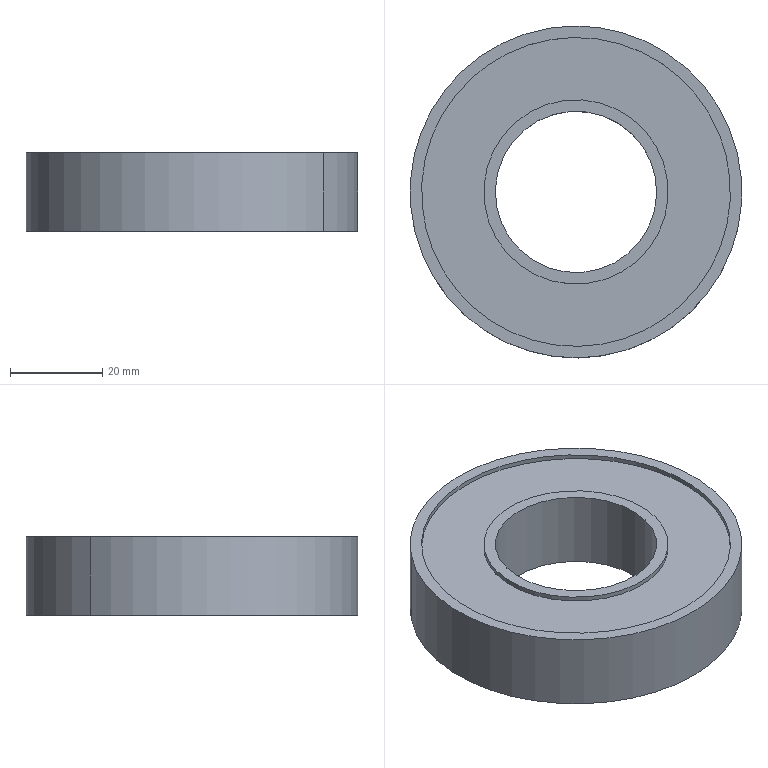Component | SolidWorks | One-wayBearing6207-1 | 1 solid | 18 faces | box 72 x 72 x 17 mm | volume 48322 mm3 | cylinder 12 | plane 6 | commonest cylinder face diameters 40 x4 67 x4 35 x2 72 x2 | material A3
build123d program:
from build123d import *

# Parameters (mm, degrees)
SKETCH1_R           = 36
SKETCH1_R_2         = 17.5
BOSS_EXTRUDE1_DEPTH = 8.5
SKETCH2_R           = 33.5
SKETCH2_R_2         = 20
CUT_EXTRUDE1_DEPTH  = 1


with BuildPart() as part:
    # Sketch1 → Boss-Extrude1 (new, symmetric)
    with BuildSketch(Plane(origin=(0, 0, 0), x_dir=(1, 0, 0), z_dir=(0, 1, 0))):
        with Locations(Location((0, 0, 0), (0, 0, 270))):
            Circle(SKETCH1_R)
        with Locations(Location((0, 0, 0), (0, 0, 270))):
            Circle(SKETCH1_R_2, mode=Mode.SUBTRACT)
    extrude(amount=BOSS_EXTRUDE1_DEPTH, both=True)

    # Sketch2 → Cut-Extrude1 (cut)
    with BuildSketch(Plane(origin=(0, 8.5, 0), x_dir=(1, 0, 0), z_dir=(0, 1, 0))):
        with Locations(Location((0, 0, 0), (0, 0, 270))):
            Circle(SKETCH2_R)
        with Locations(Location((0, 0, 0), (0, 0, 270))):
            Circle(SKETCH2_R_2, mode=Mode.SUBTRACT)
    cut_extrude1 = extrude(amount=-CUT_EXTRUDE1_DEPTH, mode=Mode.SUBTRACT)

    # Mirror1: Cut-Extrude1 across plane
    add(cut_extrude1.mirror(Plane.ZX), mode=Mode.SUBTRACT)


solid = part.part

# Placed as in the assembly
solid = solid.moved(Location((733.029, 200.722, 34), (90, 0, 0)))
STEP:
#1=COLOUR_RGB('',0.7922,0.8196,0.9333);
#2=FILL_AREA_STYLE_COLOUR('',#1);
#3=FILL_AREA_STYLE('',(#2));
#4=SURFACE_STYLE_FILL_AREA(#3);
#5=SURFACE_SIDE_STYLE('',(#4));
#6=SURFACE_STYLE_USAGE(.BOTH.,#5);
#7=PRESENTATION_STYLE_ASSIGNMENT((#6));
#8=CARTESIAN_POINT('',(29.481,7.42,1.043));
#9=VERTEX_POINT('',#8);
#10=CARTESIAN_POINT('',(28.237,8.385,1.043));
#11=VERTEX_POINT('',#10);
#12=CARTESIAN_POINT('',(28.859,7.902,1.043));
#13=DIRECTION('',(0.,0.,1.));
#14=DIRECTION('',(0.7899,-0.6132,0.));
#15=AXIS2_PLACEMENT_3D('',#12,#13,#14);
#16=CIRCLE('',#15,0.7874);
#17=EDGE_CURVE('',#9,#11,#16,.T.);
#18=ORIENTED_EDGE('',*,*,#17,.F.);
#19=CARTESIAN_POINT('',(29.481,7.42,1.004));
#20=VERTEX_POINT('',#19);
#21=CARTESIAN_POINT('',(29.481,7.42,1.043));
#22=DIRECTION('',(-0.,-0.,-1.));
#23=VECTOR('',#22,39.37);
#24=LINE('',#21,#23);
#25=EDGE_CURVE('',#9,#20,#24,.T.);
#26=ORIENTED_EDGE('',*,*,#25,.T.);
#27=CARTESIAN_POINT('',(28.237,8.385,1.004));
#28=VERTEX_POINT('',#27);
#29=CARTESIAN_POINT('',(28.859,7.902,1.004));
#30=DIRECTION('',(0.,0.,1.));
#31=DIRECTION('',(0.7899,-0.6132,0.));
#32=AXIS2_PLACEMENT_3D('',#29,#30,#31);
#33=CIRCLE('',#32,0.7874);
#34=EDGE_CURVE('',#20,#28,#33,.T.);
#35=ORIENTED_EDGE('',*,*,#34,.T.);
#36=CARTESIAN_POINT('',(28.237,8.385,1.043));
#37=DIRECTION('',(-0.,-0.,-1.));
#38=VECTOR('',#37,39.37);
#39=LINE('',#36,#38);
#40=EDGE_CURVE('',#11,#28,#39,.T.);
#41=ORIENTED_EDGE('',*,*,#40,.F.);
#42=EDGE_LOOP('',(#18,#26,#35,#41));
#43=FACE_OUTER_BOUND('',#42,.T.);
#44=CARTESIAN_POINT('',(28.859,7.902,1.043));
#45=DIRECTION('',(-0.,-0.,-1.));
#46=DIRECTION('',(-0.7899,0.6132,0.));
#47=AXIS2_PLACEMENT_3D('',#44,#45,#46);
#48=CYLINDRICAL_SURFACE('',#47,0.7874);
#49=ADVANCED_FACE('',(#43),#48,.T.);
#50=CARTESIAN_POINT('',(27.818,8.711,1.043));
#51=VERTEX_POINT('',#50);
#52=CARTESIAN_POINT('',(29.901,7.094,1.043));
#53=VERTEX_POINT('',#52);
#54=CARTESIAN_POINT('',(28.859,7.902,1.043));
#55=DIRECTION('',(0.,0.,1.));
#56=DIRECTION('',(0.7899,-0.6132,0.));
#57=AXIS2_PLACEMENT_3D('',#54,#55,#56);
#58=CIRCLE('',#57,1.319);
#59=EDGE_CURVE('',#51,#53,#58,.T.);
#60=ORIENTED_EDGE('',*,*,#59,.T.);
#61=CARTESIAN_POINT('',(29.901,7.094,1.004));
#62=VERTEX_POINT('',#61);
#63=CARTESIAN_POINT('',(29.901,7.094,1.043));
#64=DIRECTION('',(-0.,-0.,-1.));
#65=VECTOR('',#64,39.37);
#66=LINE('',#63,#65);
#67=EDGE_CURVE('',#53,#62,#66,.T.);
#68=ORIENTED_EDGE('',*,*,#67,.T.);
#69=CARTESIAN_POINT('',(27.818,8.711,1.004));
#70=VERTEX_POINT('',#69);
#71=CARTESIAN_POINT('',(28.859,7.902,1.004));
#72=DIRECTION('',(0.,0.,1.));
#73=DIRECTION('',(0.7899,-0.6132,0.));
#74=AXIS2_PLACEMENT_3D('',#71,#72,#73);
#75=CIRCLE('',#74,1.319);
#76=EDGE_CURVE('',#70,#62,#75,.T.);
#77=ORIENTED_EDGE('',*,*,#76,.F.);
#78=CARTESIAN_POINT('',(27.818,8.711,1.043));
#79=DIRECTION('',(-0.,-0.,-1.));
#80=VECTOR('',#79,39.37);
#81=LINE('',#78,#80);
#82=EDGE_CURVE('',#51,#70,#81,.T.);
#83=ORIENTED_EDGE('',*,*,#82,.F.);
#84=EDGE_LOOP('',(#60,#68,#77,#83));
#85=FACE_OUTER_BOUND('',#84,.T.);
#86=CARTESIAN_POINT('',(28.859,7.902,1.043));
#87=DIRECTION('',(-0.,-0.,-1.));
#88=DIRECTION('',(-0.7899,0.6132,0.));
#89=AXIS2_PLACEMENT_3D('',#86,#87,#88);
#90=CYLINDRICAL_SURFACE('',#89,1.319);
#91=ADVANCED_FACE('',(#85),#90,.F.);
#92=CARTESIAN_POINT('',(29.481,7.42,1.634));
#93=VERTEX_POINT('',#92);
#94=CARTESIAN_POINT('',(28.237,8.385,1.634));
#95=VERTEX_POINT('',#94);
#96=CARTESIAN_POINT('',(28.859,7.902,1.634));
#97=DIRECTION('',(0.,0.,1.));
#98=DIRECTION('',(0.7899,-0.6132,0.));
#99=AXIS2_PLACEMENT_3D('',#96,#97,#98);
#100=CIRCLE('',#99,0.7874);
#101=EDGE_CURVE('',#93,#95,#100,.T.);
#102=ORIENTED_EDGE('',*,*,#101,.T.);
#103=CARTESIAN_POINT('',(28.237,8.385,1.673));
#104=VERTEX_POINT('',#103);
#105=CARTESIAN_POINT('',(28.237,8.385,1.634));
#106=DIRECTION('',(0.,0.,1.));
#107=VECTOR('',#106,39.37);
#108=LINE('',#105,#107);
#109=EDGE_CURVE('',#95,#104,#108,.T.);
#110=ORIENTED_EDGE('',*,*,#109,.T.);
#111=CARTESIAN_POINT('',(29.481,7.42,1.673));
#112=VERTEX_POINT('',#111);
#113=CARTESIAN_POINT('',(28.859,7.902,1.673));
#114=DIRECTION('',(0.,0.,1.));
#115=DIRECTION('',(0.7899,-0.6132,0.));
#116=AXIS2_PLACEMENT_3D('',#113,#114,#115);
#117=CIRCLE('',#116,0.7874);
#118=EDGE_CURVE('',#112,#104,#117,.T.);
#119=ORIENTED_EDGE('',*,*,#118,.F.);
#120=CARTESIAN_POINT('',(29.481,7.42,1.634));
#121=DIRECTION('',(0.,0.,1.));
#122=VECTOR('',#121,39.37);
#123=LINE('',#120,#122);
#124=EDGE_CURVE('',#93,#112,#123,.T.);
#125=ORIENTED_EDGE('',*,*,#124,.F.);
#126=EDGE_LOOP('',(#102,#110,#119,#125));
#127=FACE_OUTER_BOUND('',#126,.T.);
#128=CARTESIAN_POINT('',(28.859,7.902,1.634));
#129=DIRECTION('',(0.,0.,1.));
#130=DIRECTION('',(0.7899,-0.6132,0.));
#131=AXIS2_PLACEMENT_3D('',#128,#129,#130);
#132=CYLINDRICAL_SURFACE('',#131,0.7874);
#133=ADVANCED_FACE('',(#127),#132,.T.);
#134=CARTESIAN_POINT('',(27.818,8.711,1.634));
#135=VERTEX_POINT('',#134);
#136=CARTESIAN_POINT('',(29.901,7.094,1.634));
#137=VERTEX_POINT('',#136);
#138=CARTESIAN_POINT('',(28.859,7.902,1.634));
#139=DIRECTION('',(0.,0.,1.));
#140=DIRECTION('',(0.7899,-0.6132,0.));
#141=AXIS2_PLACEMENT_3D('',#138,#139,#140);
#142=CIRCLE('',#141,1.319);
#143=EDGE_CURVE('',#135,#137,#142,.T.);
#144=ORIENTED_EDGE('',*,*,#143,.F.);
#145=CARTESIAN_POINT('',(27.818,8.711,1.673));
#146=VERTEX_POINT('',#145);
#147=CARTESIAN_POINT('',(27.818,8.711,1.634));
#148=DIRECTION('',(0.,0.,1.));
#149=VECTOR('',#148,39.37);
#150=LINE('',#147,#149);
#151=EDGE_CURVE('',#135,#146,#150,.T.);
#152=ORIENTED_EDGE('',*,*,#151,.T.);
#153=CARTESIAN_POINT('',(29.901,7.094,1.673));
#154=VERTEX_POINT('',#153);
#155=CARTESIAN_POINT('',(28.859,7.902,1.673));
#156=DIRECTION('',(0.,0.,1.));
#157=DIRECTION('',(0.7899,-0.6132,0.));
#158=AXIS2_PLACEMENT_3D('',#155,#156,#157);
#159=CIRCLE('',#158,1.319);
#160=EDGE_CURVE('',#146,#154,#159,.T.);
#161=ORIENTED_EDGE('',*,*,#160,.T.);
#162=CARTESIAN_POINT('',(29.901,7.094,1.634));
#163=DIRECTION('',(0.,0.,1.));
#164=VECTOR('',#163,39.37);
#165=LINE('',#162,#164);
#166=EDGE_CURVE('',#137,#154,#165,.T.);
#167=ORIENTED_EDGE('',*,*,#166,.F.);
#168=EDGE_LOOP('',(#144,#152,#161,#167));
#169=FACE_OUTER_BOUND('',#168,.T.);
#170=CARTESIAN_POINT('',(28.859,7.902,1.634));
#171=DIRECTION('',(0.,0.,1.));
#172=DIRECTION('',(0.7899,-0.6132,0.));
#173=AXIS2_PLACEMENT_3D('',#170,#171,#172);
#174=CYLINDRICAL_SURFACE('',#173,1.319);
#175=ADVANCED_FACE('',(#169),#174,.F.);
#176=CARTESIAN_POINT('',(28.315,8.325,1.673));
#177=VERTEX_POINT('',#176);
#178=CARTESIAN_POINT('',(29.404,7.48,1.673));
#179=VERTEX_POINT('',#178);
#180=CARTESIAN_POINT('',(28.859,7.902,1.673));
#181=DIRECTION('',(0.,0.,1.));
#182=DIRECTION('',(0.7899,-0.6132,0.));
#183=AXIS2_PLACEMENT_3D('',#180,#181,#182);
#184=CIRCLE('',#183,0.689);
#185=EDGE_CURVE('',#177,#179,#184,.T.);
#186=ORIENTED_EDGE('',*,*,#185,.T.);
#187=CARTESIAN_POINT('',(29.404,7.48,1.004));
#188=VERTEX_POINT('',#187);
#189=CARTESIAN_POINT('',(29.404,7.48,1.673));
#190=DIRECTION('',(-0.,-0.,-1.));
#191=VECTOR('',#190,39.37);
#192=LINE('',#189,#191);
#193=EDGE_CURVE('',#179,#188,#192,.T.);
#194=ORIENTED_EDGE('',*,*,#193,.T.);
#195=CARTESIAN_POINT('',(28.315,8.325,1.004));
#196=VERTEX_POINT('',#195);
#197=CARTESIAN_POINT('',(28.859,7.902,1.004));
#198=DIRECTION('',(0.,0.,1.));
#199=DIRECTION('',(0.7899,-0.6132,0.));
#200=AXIS2_PLACEMENT_3D('',#197,#198,#199);
#201=CIRCLE('',#200,0.689);
#202=EDGE_CURVE('',#196,#188,#201,.T.);
#203=ORIENTED_EDGE('',*,*,#202,.F.);
#204=CARTESIAN_POINT('',(28.315,8.325,1.673));
#205=DIRECTION('',(-0.,-0.,-1.));
#206=VECTOR('',#205,39.37);
#207=LINE('',#204,#206);
#208=EDGE_CURVE('',#177,#196,#207,.T.);
#209=ORIENTED_EDGE('',*,*,#208,.F.);
#210=EDGE_LOOP('',(#186,#194,#203,#209));
#211=FACE_OUTER_BOUND('',#210,.T.);
#212=CARTESIAN_POINT('',(28.859,7.902,1.673));
#213=DIRECTION('',(-0.,-0.,-1.));
#214=DIRECTION('',(-0.7899,0.6132,0.));
#215=AXIS2_PLACEMENT_3D('',#212,#213,#214);
#216=CYLINDRICAL_SURFACE('',#215,0.689);
#217=ADVANCED_FACE('',(#211),#216,.F.);
#218=CARTESIAN_POINT('',(29.979,7.033,1.673));
#219=VERTEX_POINT('',#218);
#220=CARTESIAN_POINT('',(27.74,8.772,1.673));
#221=VERTEX_POINT('',#220);
#222=CARTESIAN_POINT('',(28.859,7.902,1.673));
#223=DIRECTION('',(0.,0.,1.));
#224=DIRECTION('',(0.7899,-0.6132,0.));
#225=AXIS2_PLACEMENT_3D('',#222,#223,#224);
#226=CIRCLE('',#225,1.417);
#227=EDGE_CURVE('',#219,#221,#226,.T.);
#228=ORIENTED_EDGE('',*,*,#227,.F.);
#229=CARTESIAN_POINT('',(29.979,7.033,1.004));
#230=VERTEX_POINT('',#229);
#231=CARTESIAN_POINT('',(29.979,7.033,1.673));
#232=DIRECTION('',(-0.,-0.,-1.));
#233=VECTOR('',#232,39.37);
#234=LINE('',#231,#233);
#235=EDGE_CURVE('',#219,#230,#234,.T.);
#236=ORIENTED_EDGE('',*,*,#235,.T.);
#237=CARTESIAN_POINT('',(27.74,8.772,1.004));
#238=VERTEX_POINT('',#237);
#239=CARTESIAN_POINT('',(28.859,7.902,1.004));
#240=DIRECTION('',(0.,0.,1.));
#241=DIRECTION('',(0.7899,-0.6132,0.));
#242=AXIS2_PLACEMENT_3D('',#239,#240,#241);
#243=CIRCLE('',#242,1.417);
#244=EDGE_CURVE('',#230,#238,#243,.T.);
#245=ORIENTED_EDGE('',*,*,#244,.T.);
#246=CARTESIAN_POINT('',(27.74,8.772,1.673));
#247=DIRECTION('',(-0.,-0.,-1.));
#248=VECTOR('',#247,39.37);
#249=LINE('',#246,#248);
#250=EDGE_CURVE('',#221,#238,#249,.T.);
#251=ORIENTED_EDGE('',*,*,#250,.F.);
#252=EDGE_LOOP('',(#228,#236,#245,#251));
#253=FACE_OUTER_BOUND('',#252,.T.);
#254=CARTESIAN_POINT('',(28.859,7.902,1.673));
#255=DIRECTION('',(-0.,-0.,-1.));
#256=DIRECTION('',(-0.7899,0.6132,0.));
#257=AXIS2_PLACEMENT_3D('',#254,#255,#256);
#258=CYLINDRICAL_SURFACE('',#257,1.417);
#259=ADVANCED_FACE('',(#253),#258,.T.);
#260=ORIENTED_EDGE('',*,*,#202,.T.);
#261=CARTESIAN_POINT('',(28.859,7.902,1.004));
#262=DIRECTION('',(0.,0.,1.));
#263=DIRECTION('',(0.7899,-0.6132,0.));
#264=AXIS2_PLACEMENT_3D('',#261,#262,#263);
#265=CIRCLE('',#264,0.689);
#266=EDGE_CURVE('',#188,#196,#265,.T.);
#267=ORIENTED_EDGE('',*,*,#266,.T.);
#268=EDGE_LOOP('',(#260,#267));
#269=FACE_BOUND('',#268,.T.);
#270=CARTESIAN_POINT('',(28.859,7.902,1.004));
#271=DIRECTION('',(0.,0.,1.));
#272=DIRECTION('',(0.7899,-0.6132,0.));
#273=AXIS2_PLACEMENT_3D('',#270,#271,#272);
#274=CIRCLE('',#273,0.7874);
#275=EDGE_CURVE('',#28,#20,#274,.T.);
#276=ORIENTED_EDGE('',*,*,#275,.F.);
#277=ORIENTED_EDGE('',*,*,#34,.F.);
#278=EDGE_LOOP('',(#276,#277));
#279=FACE_OUTER_BOUND('',#278,.T.);
#280=CARTESIAN_POINT('',(28.859,7.902,1.004));
#281=DIRECTION('',(0.,0.,1.));
#282=DIRECTION('',(0.7899,-0.6132,0.));
#283=AXIS2_PLACEMENT_3D('',#280,#281,#282);
#284=PLANE('',#283);
#285=ADVANCED_FACE('',(#269,#279),#284,.F.);
#286=ORIENTED_EDGE('',*,*,#185,.F.);
#287=CARTESIAN_POINT('',(28.859,7.902,1.673));
#288=DIRECTION('',(0.,0.,1.));
#289=DIRECTION('',(0.7899,-0.6132,0.));
#290=AXIS2_PLACEMENT_3D('',#287,#288,#289);
#291=CIRCLE('',#290,0.689);
#292=EDGE_CURVE('',#179,#177,#291,.T.);
#293=ORIENTED_EDGE('',*,*,#292,.F.);
#294=EDGE_LOOP('',(#286,#293));
#295=FACE_BOUND('',#294,.T.);
#296=ORIENTED_EDGE('',*,*,#118,.T.);
#297=CARTESIAN_POINT('',(28.859,7.902,1.673));
#298=DIRECTION('',(0.,0.,1.));
#299=DIRECTION('',(0.7899,-0.6132,0.));
#300=AXIS2_PLACEMENT_3D('',#297,#298,#299);
#301=CIRCLE('',#300,0.7874);
#302=EDGE_CURVE('',#104,#112,#301,.T.);
#303=ORIENTED_EDGE('',*,*,#302,.T.);
#304=EDGE_LOOP('',(#296,#303));
#305=FACE_OUTER_BOUND('',#304,.T.);
#306=CARTESIAN_POINT('',(28.859,7.902,1.673));
#307=DIRECTION('',(0.,0.,1.));
#308=DIRECTION('',(0.7899,-0.6132,0.));
#309=AXIS2_PLACEMENT_3D('',#306,#307,#308);
#310=PLANE('',#309);
#311=ADVANCED_FACE('',(#295,#305),#310,.T.);
#312=CARTESIAN_POINT('',(28.859,7.902,1.673));
#313=DIRECTION('',(0.,0.,1.));
#314=DIRECTION('',(0.7899,-0.6132,0.));
#315=AXIS2_PLACEMENT_3D('',#312,#313,#314);
#316=CIRCLE('',#315,1.319);
#317=EDGE_CURVE('',#154,#146,#316,.T.);
#318=ORIENTED_EDGE('',*,*,#317,.F.);
#319=ORIENTED_EDGE('',*,*,#160,.F.);
#320=EDGE_LOOP('',(#318,#319));
#321=FACE_BOUND('',#320,.T.);
#322=CARTESIAN_POINT('',(28.859,7.902,1.673));
#323=DIRECTION('',(0.,0.,1.));
#324=DIRECTION('',(0.7899,-0.6132,0.));
#325=AXIS2_PLACEMENT_3D('',#322,#323,#324);
#326=CIRCLE('',#325,1.417);
#327=EDGE_CURVE('',#221,#219,#326,.T.);
#328=ORIENTED_EDGE('',*,*,#327,.T.);
#329=ORIENTED_EDGE('',*,*,#227,.T.);
#330=EDGE_LOOP('',(#328,#329));
#331=FACE_OUTER_BOUND('',#330,.T.);
#332=CARTESIAN_POINT('',(28.859,7.902,1.673));
#333=DIRECTION('',(0.,0.,1.));
#334=DIRECTION('',(0.7899,-0.6132,0.));
#335=AXIS2_PLACEMENT_3D('',#332,#333,#334);
#336=PLANE('',#335);
#337=ADVANCED_FACE('',(#321,#331),#336,.T.);
#338=ORIENTED_EDGE('',*,*,#76,.T.);
#339=CARTESIAN_POINT('',(28.859,7.902,1.004));
#340=DIRECTION('',(0.,0.,1.));
#341=DIRECTION('',(0.7899,-0.6132,0.));
#342=AXIS2_PLACEMENT_3D('',#339,#340,#341);
#343=CIRCLE('',#342,1.319);
#344=EDGE_CURVE('',#62,#70,#343,.T.);
#345=ORIENTED_EDGE('',*,*,#344,.T.);
#346=EDGE_LOOP('',(#338,#345));
#347=FACE_BOUND('',#346,.T.);
#348=CARTESIAN_POINT('',(28.859,7.902,1.004));
#349=DIRECTION('',(0.,0.,1.));
#350=DIRECTION('',(0.7899,-0.6132,0.));
#351=AXIS2_PLACEMENT_3D('',#348,#349,#350);
#352=CIRCLE('',#351,1.417);
#353=EDGE_CURVE('',#238,#230,#352,.T.);
#354=ORIENTED_EDGE('',*,*,#353,.F.);
#355=ORIENTED_EDGE('',*,*,#244,.F.);
#356=EDGE_LOOP('',(#354,#355));
#357=FACE_OUTER_BOUND('',#356,.T.);
#358=CARTESIAN_POINT('',(28.859,7.902,1.004));
#359=DIRECTION('',(0.,0.,1.));
#360=DIRECTION('',(0.7899,-0.6132,0.));
#361=AXIS2_PLACEMENT_3D('',#358,#359,#360);
#362=PLANE('',#361);
#363=ADVANCED_FACE('',(#347,#357),#362,.F.);
#364=ORIENTED_EDGE('',*,*,#235,.F.);
#365=ORIENTED_EDGE('',*,*,#327,.F.);
#366=ORIENTED_EDGE('',*,*,#250,.T.);
#367=ORIENTED_EDGE('',*,*,#353,.T.);
#368=EDGE_LOOP('',(#364,#365,#366,#367));
#369=FACE_OUTER_BOUND('',#368,.T.);
#370=CARTESIAN_POINT('',(28.859,7.902,1.673));
#371=DIRECTION('',(-0.,-0.,-1.));
#372=DIRECTION('',(-0.7899,0.6132,0.));
#373=AXIS2_PLACEMENT_3D('',#370,#371,#372);
#374=CYLINDRICAL_SURFACE('',#373,1.417);
#375=ADVANCED_FACE('',(#369),#374,.T.);
#376=ORIENTED_EDGE('',*,*,#193,.F.);
#377=ORIENTED_EDGE('',*,*,#292,.T.);
#378=ORIENTED_EDGE('',*,*,#208,.T.);
#379=ORIENTED_EDGE('',*,*,#266,.F.);
#380=EDGE_LOOP('',(#376,#377,#378,#379));
#381=FACE_OUTER_BOUND('',#380,.T.);
#382=CARTESIAN_POINT('',(28.859,7.902,1.673));
#383=DIRECTION('',(-0.,-0.,-1.));
#384=DIRECTION('',(-0.7899,0.6132,0.));
#385=AXIS2_PLACEMENT_3D('',#382,#383,#384);
#386=CYLINDRICAL_SURFACE('',#385,0.689);
#387=ADVANCED_FACE('',(#381),#386,.F.);
#388=ORIENTED_EDGE('',*,*,#151,.F.);
#389=CARTESIAN_POINT('',(28.859,7.902,1.634));
#390=DIRECTION('',(0.,0.,1.));
#391=DIRECTION('',(0.7899,-0.6132,0.));
#392=AXIS2_PLACEMENT_3D('',#389,#390,#391);
#393=CIRCLE('',#392,1.319);
#394=EDGE_CURVE('',#137,#135,#393,.T.);
#395=ORIENTED_EDGE('',*,*,#394,.F.);
#396=ORIENTED_EDGE('',*,*,#166,.T.);
#397=ORIENTED_EDGE('',*,*,#317,.T.);
#398=EDGE_LOOP('',(#388,#395,#396,#397));
#399=FACE_OUTER_BOUND('',#398,.T.);
#400=CARTESIAN_POINT('',(28.859,7.902,1.634));
#401=DIRECTION('',(0.,0.,1.));
#402=DIRECTION('',(0.7899,-0.6132,0.));
#403=AXIS2_PLACEMENT_3D('',#400,#401,#402);
#404=CYLINDRICAL_SURFACE('',#403,1.319);
#405=ADVANCED_FACE('',(#399),#404,.F.);
#406=ORIENTED_EDGE('',*,*,#101,.F.);
#407=CARTESIAN_POINT('',(28.859,7.902,1.634));
#408=DIRECTION('',(0.,0.,1.));
#409=DIRECTION('',(0.7899,-0.6132,0.));
#410=AXIS2_PLACEMENT_3D('',#407,#408,#409);
#411=CIRCLE('',#410,0.7874);
#412=EDGE_CURVE('',#95,#93,#411,.T.);
#413=ORIENTED_EDGE('',*,*,#412,.F.);
#414=EDGE_LOOP('',(#406,#413));
#415=FACE_BOUND('',#414,.T.);
#416=ORIENTED_EDGE('',*,*,#394,.T.);
#417=ORIENTED_EDGE('',*,*,#143,.T.);
#418=EDGE_LOOP('',(#416,#417));
#419=FACE_OUTER_BOUND('',#418,.T.);
#420=CARTESIAN_POINT('',(28.859,7.902,1.634));
#421=DIRECTION('',(0.,0.,1.));
#422=DIRECTION('',(0.7899,-0.6132,0.));
#423=AXIS2_PLACEMENT_3D('',#420,#421,#422);
#424=PLANE('',#423);
#425=ADVANCED_FACE('',(#415,#419),#424,.T.);
#426=ORIENTED_EDGE('',*,*,#109,.F.);
#427=ORIENTED_EDGE('',*,*,#412,.T.);
#428=ORIENTED_EDGE('',*,*,#124,.T.);
#429=ORIENTED_EDGE('',*,*,#302,.F.);
#430=EDGE_LOOP('',(#426,#427,#428,#429));
#431=FACE_OUTER_BOUND('',#430,.T.);
#432=CARTESIAN_POINT('',(28.859,7.902,1.634));
#433=DIRECTION('',(0.,0.,1.));
#434=DIRECTION('',(0.7899,-0.6132,0.));
#435=AXIS2_PLACEMENT_3D('',#432,#433,#434);
#436=CYLINDRICAL_SURFACE('',#435,0.7874);
#437=ADVANCED_FACE('',(#431),#436,.T.);
#438=ORIENTED_EDGE('',*,*,#59,.F.);
#439=CARTESIAN_POINT('',(28.859,7.902,1.043));
#440=DIRECTION('',(0.,0.,1.));
#441=DIRECTION('',(0.7899,-0.6132,0.));
#442=AXIS2_PLACEMENT_3D('',#439,#440,#441);
#443=CIRCLE('',#442,1.319);
#444=EDGE_CURVE('',#53,#51,#443,.T.);
#445=ORIENTED_EDGE('',*,*,#444,.F.);
#446=EDGE_LOOP('',(#438,#445));
#447=FACE_OUTER_BOUND('',#446,.T.);
#448=CARTESIAN_POINT('',(28.859,7.902,1.043));
#449=DIRECTION('',(0.,0.,1.));
#450=DIRECTION('',(0.7899,-0.6132,0.));
#451=AXIS2_PLACEMENT_3D('',#448,#449,#450);
#452=CIRCLE('',#451,0.7874);
#453=EDGE_CURVE('',#11,#9,#452,.T.);
#454=ORIENTED_EDGE('',*,*,#453,.T.);
#455=ORIENTED_EDGE('',*,*,#17,.T.);
#456=EDGE_LOOP('',(#454,#455));
#457=FACE_BOUND('',#456,.T.);
#458=CARTESIAN_POINT('',(28.859,7.902,1.043));
#459=DIRECTION('',(-0.,-0.,-1.));
#460=DIRECTION('',(0.7899,-0.6132,0.));
#461=AXIS2_PLACEMENT_3D('',#458,#459,#460);
#462=PLANE('',#461);
#463=ADVANCED_FACE('',(#447,#457),#462,.T.);
#464=ORIENTED_EDGE('',*,*,#67,.F.);
#465=ORIENTED_EDGE('',*,*,#444,.T.);
#466=ORIENTED_EDGE('',*,*,#82,.T.);
#467=ORIENTED_EDGE('',*,*,#344,.F.);
#468=EDGE_LOOP('',(#464,#465,#466,#467));
#469=FACE_OUTER_BOUND('',#468,.T.);
#470=CARTESIAN_POINT('',(28.859,7.902,1.043));
#471=DIRECTION('',(-0.,-0.,-1.));
#472=DIRECTION('',(-0.7899,0.6132,0.));
#473=AXIS2_PLACEMENT_3D('',#470,#471,#472);
#474=CYLINDRICAL_SURFACE('',#473,1.319);
#475=ADVANCED_FACE('',(#469),#474,.F.);
#476=ORIENTED_EDGE('',*,*,#25,.F.);
#477=ORIENTED_EDGE('',*,*,#453,.F.);
#478=ORIENTED_EDGE('',*,*,#40,.T.);
#479=ORIENTED_EDGE('',*,*,#275,.T.);
#480=EDGE_LOOP('',(#476,#477,#478,#479));
#481=FACE_OUTER_BOUND('',#480,.T.);
#482=CARTESIAN_POINT('',(28.859,7.902,1.043));
#483=DIRECTION('',(-0.,-0.,-1.));
#484=DIRECTION('',(-0.7899,0.6132,0.));
#485=AXIS2_PLACEMENT_3D('',#482,#483,#484);
#486=CYLINDRICAL_SURFACE('',#485,0.7874);
#487=ADVANCED_FACE('',(#481),#486,.T.);
#488=CLOSED_SHELL('',(#49,#91,#133,#175,#217,#259,#285,#311,#337,#363,#375,#387,#405,#425,#437,#463,#475,#487));
#489=MANIFOLD_SOLID_BREP('',#488);
#490=STYLED_ITEM('',(#7),#489);
#491=(LENGTH_UNIT()NAMED_UNIT(*)SI_UNIT($,.METRE.));
#492=LENGTH_MEASURE_WITH_UNIT(LENGTH_MEASURE(0.0254),#491);
#493=DIMENSIONAL_EXPONENTS(1.,0.,0.,0.,0.,0.,0.);
#494=(CONVERSION_BASED_UNIT('',#492)LENGTH_UNIT()NAMED_UNIT(#493));
#495=UNCERTAINTY_MEASURE_WITH_UNIT(LENGTH_MEASURE(0.00001),#494,'','');
#496=(NAMED_UNIT(*)PLANE_ANGLE_UNIT()SI_UNIT($,.RADIAN.));
#497=(NAMED_UNIT(*)SI_UNIT($,.STERADIAN.)SOLID_ANGLE_UNIT());
#498=(GEOMETRIC_REPRESENTATION_CONTEXT(3)GLOBAL_UNCERTAINTY_ASSIGNED_CONTEXT((#495))GLOBAL_UNIT_ASSIGNED_CONTEXT((#494,#496,#497))REPRESENTATION_CONTEXT('',''));
#499=MECHANICAL_DESIGN_GEOMETRIC_PRESENTATION_REPRESENTATION('',(#490),#498);
#500=PRESENTATION_LAYER_ASSIGNMENT('','',(#490));
#501=CARTESIAN_POINT('',(0.,0.,0.));
#502=DIRECTION('',(0.,0.,1.));
#503=DIRECTION('',(1.,0.,0.));
#504=AXIS2_PLACEMENT_3D('',#501,#502,#503);
#505=(LENGTH_UNIT()NAMED_UNIT(*)SI_UNIT($,.METRE.));
#506=LENGTH_MEASURE_WITH_UNIT(LENGTH_MEASURE(0.0254),#505);
#507=DIMENSIONAL_EXPONENTS(1.,0.,0.,0.,0.,0.,0.);
#508=(CONVERSION_BASED_UNIT('',#506)LENGTH_UNIT()NAMED_UNIT(#507));
#509=UNCERTAINTY_MEASURE_WITH_UNIT(LENGTH_MEASURE(0.00001),#508,'','');
#510=(NAMED_UNIT(*)PLANE_ANGLE_UNIT()SI_UNIT($,.RADIAN.));
#511=(NAMED_UNIT(*)SI_UNIT($,.STERADIAN.)SOLID_ANGLE_UNIT());
#512=(GEOMETRIC_REPRESENTATION_CONTEXT(3)GLOBAL_UNCERTAINTY_ASSIGNED_CONTEXT((#509))GLOBAL_UNIT_ASSIGNED_CONTEXT((#508,#510,#511))REPRESENTATION_CONTEXT('',''));
#513=ADVANCED_BREP_SHAPE_REPRESENTATION('',(#489,#504),#512);